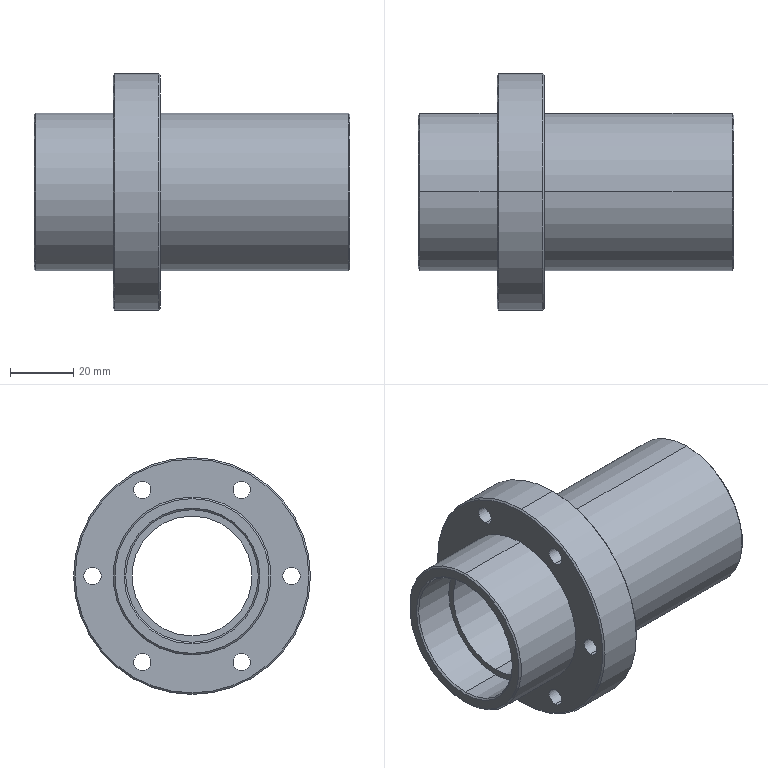Component | SolidWorks | JJDJR-3060-E-001-1 | 1 solid | 42 faces | box 100 x 75 x 75 mm | volume 110447 mm3 | cylinder 24 | cone 12 | plane 6 | commonest cylinder face diameters 5.5 x12 50 x4 42 x4 75 x2 38 x2 | material 45#
build123d program:
from build123d import *

# Parameters (mm, degrees)
CIRPATTERN1_COUNT = 6
CHAMFER1_SIZE     = 0.5
CHAMFER2_SIZE     = 0.5


with BuildPart() as part:
    # Sketch1 → Revolve1 (revolve)
    with BuildSketch(Plane.XY, mode=Mode.PRIVATE) as revolve1_sk:
        Polygon((0, 25), (25, 25), (25, 37.5), (40, 37.5), (40, 25), (100, 25), (100, 21), (86, 21), (86, 19), (14, 19), (14, 21), (0, 21), align=None)
    revolve(revolve1_sk.sketch.rotate(Axis((0, 0, 0), (1, 0, 0)), 90), axis=Axis((0, 0, 0), (1, 0, 0)))

    # Sketch2 → 5.5 _5.5_ Diameter Hole1 (revolve, cut)
    with BuildSketch(Plane(origin=(40, 31.5, 0), x_dir=(0, 0, -1), z_dir=(0, 1, 0))):
        Polygon((0, 0), (0, 16.652), (2.75, 15), (2.75, 0), align=None)
    f_5_5_5_5_diameter_hole1 = revolve(axis=Axis((46.35, 31.5, 0), (-1, 0, 0)), mode=Mode.SUBTRACT)

    # CirPattern1: 5.5 _5.5_ Diameter Hole1 ×6 about axis
    cirpattern1_axis = Axis((0, 0, 0), (1, 0, 0))
    for i in range(1, CIRPATTERN1_COUNT):
        add(f_5_5_5_5_diameter_hole1.rotate(cirpattern1_axis, i * 360 / CIRPATTERN1_COUNT), mode=Mode.SUBTRACT)

    # Chamfer1
    chamfer1_edges = [part.edges().sort_by_distance(p)[0] for p in [
        (0, 0, -25),
        (40, 0, -37.5),
        (25, 0, -37.5),
    ]]
    chamfer(chamfer1_edges, length=CHAMFER1_SIZE)

    # Chamfer2
    chamfer2_edges = [part.edges().sort_by_distance(p)[0] for p in [
        (0, 0, -21),
        (100, 0, -21),
        (100, 0, -25),
    ]]
    chamfer(chamfer2_edges, length=CHAMFER2_SIZE)


solid = part.part

# Placed as in the assembly
solid = solid.moved(Location((-103.59, -29.263, -16.52), (0, 0, 0)))